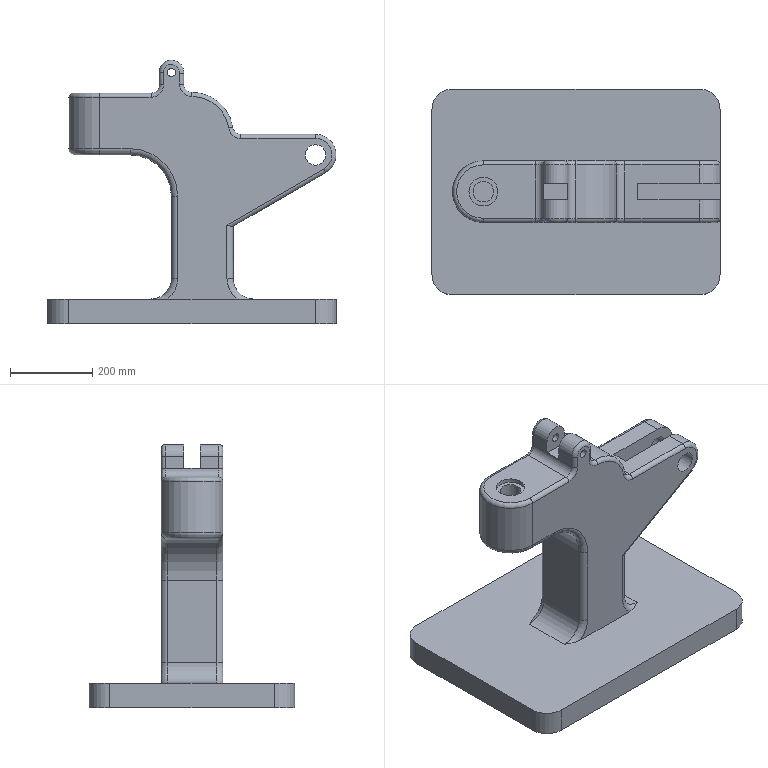Component | NX | MACHINE_BASE | 1 solid | 85 faces | volume 41953054 mm3 | cylinder 38 | plane 27 | torus 20 | commonest cylinder face diameters 20 x12 100 x8 30 x6 50 x3 40 x3 60 x2 200 x2 150 x1